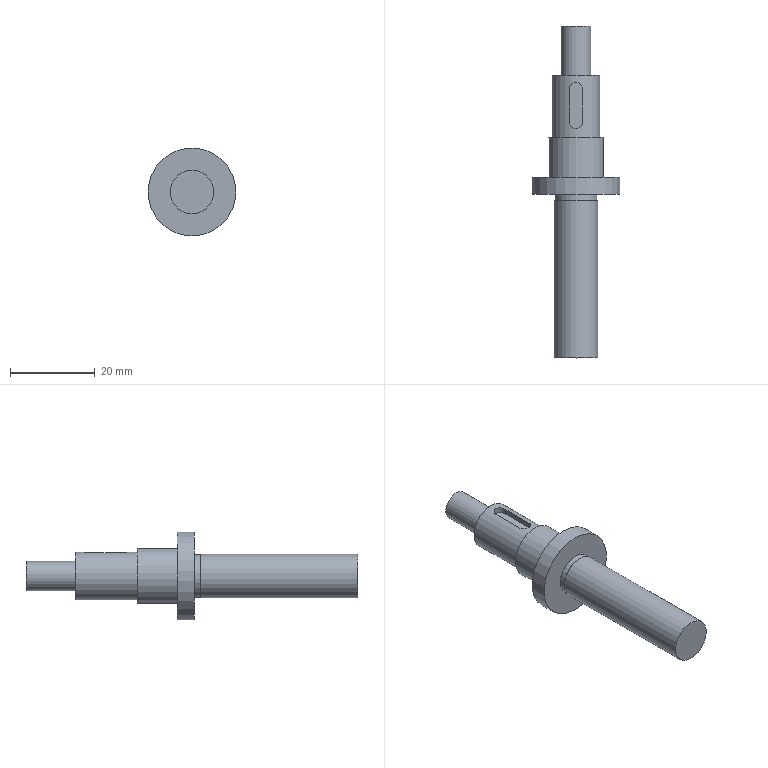Component | NX | SCREW_ROD | 1 solid | 18 faces | volume 7712 mm3 | plane 10 | cylinder 8 | commonest cylinder face diameters 3 x2 11.3 x1 10.3 x1 10 x1 20.8 x1 13 x1 6.985 x1